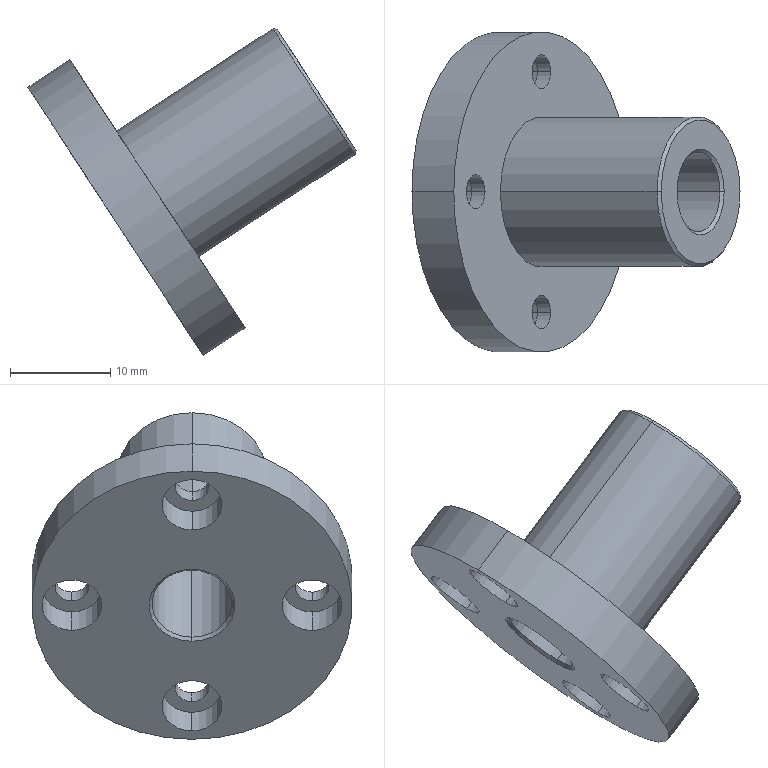Component | SolidWorks | LMF8UULinearBearing-1 | 1 solid | 35 faces | box 32.78 x 32 x 32.64 mm | volume 5725 mm3 | cylinder 22 | plane 7 | cone 6 | commonest cylinder face diameters 6 x8 3.4 x8 32 x2 8 x2 15 x2
STEP:
#1=COLOUR_RGB('',0.7922,0.8196,0.9333);
#2=FILL_AREA_STYLE_COLOUR('',#1);
#3=FILL_AREA_STYLE('',(#2));
#4=SURFACE_STYLE_FILL_AREA(#3);
#5=SURFACE_SIDE_STYLE('',(#4));
#6=SURFACE_STYLE_USAGE(.BOTH.,#5);
#7=PRESENTATION_STYLE_ASSIGNMENT((#6));
#8=CARTESIAN_POINT('',(-0.8628,2.344,0.7729));
#9=VERTEX_POINT('',#8);
#10=CARTESIAN_POINT('',(-0.6905,2.344,0.5092));
#11=VERTEX_POINT('',#10);
#12=CARTESIAN_POINT('',(-0.7767,2.344,0.6411));
#13=DIRECTION('',(0.8371,-0.,0.5471));
#14=DIRECTION('',(-0.5471,-0.0005991,0.8371));
#15=AXIS2_PLACEMENT_3D('',#12,#13,#14);
#16=CIRCLE('',#15,0.1575);
#17=EDGE_CURVE('',#9,#11,#16,.T.);
#18=ORIENTED_EDGE('',*,*,#17,.F.);
#19=CARTESIAN_POINT('',(-0.8594,2.344,0.7892));
#20=VERTEX_POINT('',#19);
#21=CARTESIAN_POINT('',(-0.8594,2.344,0.7892));
#22=DIRECTION('',(0.2051,-0.0004236,0.9787));
#23=VECTOR('',#22,39.37);
#24=LINE('',#21,#23);
#25=EDGE_CURVE('',#9,#20,#24,.T.);
#26=ORIENTED_EDGE('',*,*,#25,.T.);
#27=CARTESIAN_POINT('',(-0.6742,2.344,0.5058));
#28=VERTEX_POINT('',#27);
#29=CARTESIAN_POINT('',(-0.7668,2.344,0.6475));
#30=DIRECTION('',(-0.8371,0.,-0.5471));
#31=DIRECTION('',(-0.5471,-0.0005991,0.8371));
#32=AXIS2_PLACEMENT_3D('',#29,#30,#31);
#33=CIRCLE('',#32,0.1693);
#34=EDGE_CURVE('',#28,#20,#33,.T.);
#35=ORIENTED_EDGE('',*,*,#34,.F.);
#36=CARTESIAN_POINT('',(-0.6742,2.344,0.5058));
#37=DIRECTION('',(0.9787,0.0004236,-0.2051));
#38=VECTOR('',#37,39.37);
#39=LINE('',#36,#38);
#40=EDGE_CURVE('',#11,#28,#39,.T.);
#41=ORIENTED_EDGE('',*,*,#40,.F.);
#42=EDGE_LOOP('',(#18,#26,#35,#41));
#43=FACE_OUTER_BOUND('',#42,.T.);
#44=CARTESIAN_POINT('',(-0.7668,2.344,0.6475));
#45=DIRECTION('',(0.8371,-0.,0.5471));
#46=DIRECTION('',(0.5471,0.0005991,-0.8371));
#47=AXIS2_PLACEMENT_3D('',#44,#45,#46);
#48=CONICAL_SURFACE('',#47,0.1693,0.7854);
#49=ADVANCED_FACE('',(#43),#48,.F.);
#50=CARTESIAN_POINT('',(-0.6117,2.344,0.4102));
#51=VERTEX_POINT('',#50);
#52=CARTESIAN_POINT('',(-0.9219,2.344,0.8848));
#53=VERTEX_POINT('',#52);
#54=CARTESIAN_POINT('',(-0.7668,2.344,0.6475));
#55=DIRECTION('',(0.8371,-0.,0.5471));
#56=DIRECTION('',(-0.5471,-0.0005991,0.8371));
#57=AXIS2_PLACEMENT_3D('',#54,#55,#56);
#58=CIRCLE('',#57,0.2835);
#59=EDGE_CURVE('',#51,#53,#58,.T.);
#60=ORIENTED_EDGE('',*,*,#59,.F.);
#61=CARTESIAN_POINT('',(-0.6152,2.344,0.3939));
#62=VERTEX_POINT('',#61);
#63=CARTESIAN_POINT('',(-0.6152,2.344,0.3939));
#64=DIRECTION('',(-0.2051,0.0004236,-0.9787));
#65=VECTOR('',#64,39.37);
#66=LINE('',#63,#65);
#67=EDGE_CURVE('',#51,#62,#66,.T.);
#68=ORIENTED_EDGE('',*,*,#67,.T.);
#69=CARTESIAN_POINT('',(-0.9382,2.344,0.8882));
#70=VERTEX_POINT('',#69);
#71=CARTESIAN_POINT('',(-0.7767,2.344,0.6411));
#72=DIRECTION('',(-0.8371,0.,-0.5471));
#73=DIRECTION('',(-0.5471,-0.0005991,0.8371));
#74=AXIS2_PLACEMENT_3D('',#71,#72,#73);
#75=CIRCLE('',#74,0.2953);
#76=EDGE_CURVE('',#70,#62,#75,.T.);
#77=ORIENTED_EDGE('',*,*,#76,.F.);
#78=CARTESIAN_POINT('',(-0.9382,2.344,0.8882));
#79=DIRECTION('',(-0.9787,-0.0004236,0.2051));
#80=VECTOR('',#79,39.37);
#81=LINE('',#78,#80);
#82=EDGE_CURVE('',#53,#70,#81,.T.);
#83=ORIENTED_EDGE('',*,*,#82,.F.);
#84=EDGE_LOOP('',(#60,#68,#77,#83));
#85=FACE_OUTER_BOUND('',#84,.T.);
#86=CARTESIAN_POINT('',(-0.7767,2.344,0.6411));
#87=DIRECTION('',(-0.8371,0.,-0.5471));
#88=DIRECTION('',(-0.5471,-0.0005991,0.8371));
#89=AXIS2_PLACEMENT_3D('',#86,#87,#88);
#90=CONICAL_SURFACE('',#89,0.2953,0.7854);
#91=ADVANCED_FACE('',(#85),#90,.T.);
#92=CARTESIAN_POINT('',(-1.462,2.344,0.005266));
#93=VERTEX_POINT('',#92);
#94=CARTESIAN_POINT('',(-1.634,2.344,0.2689));
#95=VERTEX_POINT('',#94);
#96=CARTESIAN_POINT('',(-1.548,2.344,0.1371));
#97=DIRECTION('',(-0.8371,0.,-0.5471));
#98=DIRECTION('',(-0.5471,-0.0005991,0.8371));
#99=AXIS2_PLACEMENT_3D('',#96,#97,#98);
#100=CIRCLE('',#99,0.1575);
#101=EDGE_CURVE('',#93,#95,#100,.T.);
#102=ORIENTED_EDGE('',*,*,#101,.F.);
#103=CARTESIAN_POINT('',(-1.465,2.344,-0.01108));
#104=VERTEX_POINT('',#103);
#105=CARTESIAN_POINT('',(-1.462,2.344,0.005266));
#106=DIRECTION('',(-0.2051,0.0004236,-0.9787));
#107=VECTOR('',#106,39.37);
#108=LINE('',#105,#107);
#109=EDGE_CURVE('',#93,#104,#108,.T.);
#110=ORIENTED_EDGE('',*,*,#109,.T.);
#111=CARTESIAN_POINT('',(-1.65,2.344,0.2723));
#112=VERTEX_POINT('',#111);
#113=CARTESIAN_POINT('',(-1.558,2.344,0.1306));
#114=DIRECTION('',(0.8371,-0.,0.5471));
#115=DIRECTION('',(-0.5471,-0.0005991,0.8371));
#116=AXIS2_PLACEMENT_3D('',#113,#114,#115);
#117=CIRCLE('',#116,0.1693);
#118=EDGE_CURVE('',#112,#104,#117,.T.);
#119=ORIENTED_EDGE('',*,*,#118,.F.);
#120=CARTESIAN_POINT('',(-1.634,2.344,0.2689));
#121=DIRECTION('',(-0.9787,-0.0004236,0.2051));
#122=VECTOR('',#121,39.37);
#123=LINE('',#120,#122);
#124=EDGE_CURVE('',#95,#112,#123,.T.);
#125=ORIENTED_EDGE('',*,*,#124,.F.);
#126=EDGE_LOOP('',(#102,#110,#119,#125));
#127=FACE_OUTER_BOUND('',#126,.T.);
#128=CARTESIAN_POINT('',(-1.548,2.344,0.1371));
#129=DIRECTION('',(-0.8371,0.,-0.5471));
#130=DIRECTION('',(-0.5471,-0.0005991,0.8371));
#131=AXIS2_PLACEMENT_3D('',#128,#129,#130);
#132=CONICAL_SURFACE('',#131,0.1575,0.7854);
#133=ADVANCED_FACE('',(#127),#132,.F.);
#134=CARTESIAN_POINT('',(-1.381,2.817,0.1052));
#135=VERTEX_POINT('',#134);
#136=CARTESIAN_POINT('',(-1.51,2.817,0.303));
#137=VERTEX_POINT('',#136);
#138=CARTESIAN_POINT('',(-1.446,2.817,0.2041));
#139=DIRECTION('',(-0.8371,0.,-0.5471));
#140=DIRECTION('',(-0.5471,-0.0005991,0.8371));
#141=AXIS2_PLACEMENT_3D('',#138,#139,#140);
#142=CIRCLE('',#141,0.1181);
#143=EDGE_CURVE('',#135,#137,#142,.T.);
#144=ORIENTED_EDGE('',*,*,#143,.F.);
#145=CARTESIAN_POINT('',(-1.493,2.817,0.032));
#146=VERTEX_POINT('',#145);
#147=CARTESIAN_POINT('',(-1.493,2.817,0.032));
#148=DIRECTION('',(-0.8371,0.,-0.5471));
#149=VECTOR('',#148,39.37);
#150=LINE('',#147,#149);
#151=EDGE_CURVE('',#135,#146,#150,.T.);
#152=ORIENTED_EDGE('',*,*,#151,.T.);
#153=CARTESIAN_POINT('',(-1.623,2.817,0.2297));
#154=VERTEX_POINT('',#153);
#155=CARTESIAN_POINT('',(-1.558,2.817,0.1309));
#156=DIRECTION('',(-0.8371,0.,-0.5471));
#157=DIRECTION('',(-0.5471,-0.0005991,0.8371));
#158=AXIS2_PLACEMENT_3D('',#155,#156,#157);
#159=CIRCLE('',#158,0.1181);
#160=EDGE_CURVE('',#146,#154,#159,.T.);
#161=ORIENTED_EDGE('',*,*,#160,.T.);
#162=CARTESIAN_POINT('',(-1.623,2.817,0.2297));
#163=DIRECTION('',(-0.8371,0.,-0.5471));
#164=VECTOR('',#163,39.37);
#165=LINE('',#162,#164);
#166=EDGE_CURVE('',#137,#154,#165,.T.);
#167=ORIENTED_EDGE('',*,*,#166,.F.);
#168=EDGE_LOOP('',(#144,#152,#161,#167));
#169=FACE_OUTER_BOUND('',#168,.T.);
#170=CARTESIAN_POINT('',(-1.558,2.817,0.1309));
#171=DIRECTION('',(-0.8371,0.,-0.5471));
#172=DIRECTION('',(-0.5471,-0.0005991,0.8371));
#173=AXIS2_PLACEMENT_3D('',#170,#171,#172);
#174=CYLINDRICAL_SURFACE('',#173,0.1181);
#175=ADVANCED_FACE('',(#169),#174,.F.);
#176=CARTESIAN_POINT('',(-1.357,2.817,0.1825));
#177=VERTEX_POINT('',#176);
#178=CARTESIAN_POINT('',(-1.43,2.817,0.2946));
#179=VERTEX_POINT('',#178);
#180=CARTESIAN_POINT('',(-1.393,2.817,0.2386));
#181=DIRECTION('',(-0.8371,0.,-0.5471));
#182=DIRECTION('',(-0.5471,-0.0005991,0.8371));
#183=AXIS2_PLACEMENT_3D('',#180,#181,#182);
#184=CIRCLE('',#183,0.06693);
#185=EDGE_CURVE('',#177,#179,#184,.T.);
#186=ORIENTED_EDGE('',*,*,#185,.F.);
#187=CARTESIAN_POINT('',(-1.409,2.817,0.1481));
#188=VERTEX_POINT('',#187);
#189=CARTESIAN_POINT('',(-1.521,2.817,0.07484));
#190=DIRECTION('',(-0.8371,0.,-0.5471));
#191=VECTOR('',#190,39.37);
#192=LINE('',#189,#191);
#193=EDGE_CURVE('',#177,#188,#192,.T.);
#194=ORIENTED_EDGE('',*,*,#193,.T.);
#195=CARTESIAN_POINT('',(-1.482,2.817,0.2601));
#196=VERTEX_POINT('',#195);
#197=CARTESIAN_POINT('',(-1.446,2.817,0.2041));
#198=DIRECTION('',(-0.8371,0.,-0.5471));
#199=DIRECTION('',(-0.5471,-0.0005991,0.8371));
#200=AXIS2_PLACEMENT_3D('',#197,#198,#199);
#201=CIRCLE('',#200,0.06693);
#202=EDGE_CURVE('',#188,#196,#201,.T.);
#203=ORIENTED_EDGE('',*,*,#202,.T.);
#204=CARTESIAN_POINT('',(-1.595,2.817,0.1869));
#205=DIRECTION('',(-0.8371,0.,-0.5471));
#206=VECTOR('',#205,39.37);
#207=LINE('',#204,#206);
#208=EDGE_CURVE('',#179,#196,#207,.T.);
#209=ORIENTED_EDGE('',*,*,#208,.F.);
#210=EDGE_LOOP('',(#186,#194,#203,#209));
#211=FACE_OUTER_BOUND('',#210,.T.);
#212=CARTESIAN_POINT('',(-1.558,2.817,0.1309));
#213=DIRECTION('',(-0.8371,0.,-0.5471));
#214=DIRECTION('',(-0.5471,-0.0005991,0.8371));
#215=AXIS2_PLACEMENT_3D('',#212,#213,#214);
#216=CYLINDRICAL_SURFACE('',#215,0.06693);
#217=ADVANCED_FACE('',(#211),#216,.F.);
#218=CARTESIAN_POINT('',(-1.123,2.345,-0.2905));
#219=VERTEX_POINT('',#218);
#220=CARTESIAN_POINT('',(-1.252,2.345,-0.09275));
#221=VERTEX_POINT('',#220);
#222=CARTESIAN_POINT('',(-1.187,2.345,-0.1916));
#223=DIRECTION('',(-0.8371,0.,-0.5471));
#224=DIRECTION('',(-0.5471,-0.0005991,0.8371));
#225=AXIS2_PLACEMENT_3D('',#222,#223,#224);
#226=CIRCLE('',#225,0.1181);
#227=EDGE_CURVE('',#219,#221,#226,.T.);
#228=ORIENTED_EDGE('',*,*,#227,.F.);
#229=CARTESIAN_POINT('',(-1.235,2.345,-0.3637));
#230=VERTEX_POINT('',#229);
#231=CARTESIAN_POINT('',(-1.235,2.345,-0.3637));
#232=DIRECTION('',(-0.8371,0.,-0.5471));
#233=VECTOR('',#232,39.37);
#234=LINE('',#231,#233);
#235=EDGE_CURVE('',#219,#230,#234,.T.);
#236=ORIENTED_EDGE('',*,*,#235,.T.);
#237=CARTESIAN_POINT('',(-1.364,2.345,-0.166));
#238=VERTEX_POINT('',#237);
#239=CARTESIAN_POINT('',(-1.299,2.345,-0.2648));
#240=DIRECTION('',(-0.8371,0.,-0.5471));
#241=DIRECTION('',(-0.5471,-0.0005991,0.8371));
#242=AXIS2_PLACEMENT_3D('',#239,#240,#241);
#243=CIRCLE('',#242,0.1181);
#244=EDGE_CURVE('',#230,#238,#243,.T.);
#245=ORIENTED_EDGE('',*,*,#244,.T.);
#246=CARTESIAN_POINT('',(-1.364,2.345,-0.166));
#247=DIRECTION('',(-0.8371,0.,-0.5471));
#248=VECTOR('',#247,39.37);
#249=LINE('',#246,#248);
#250=EDGE_CURVE('',#221,#238,#249,.T.);
#251=ORIENTED_EDGE('',*,*,#250,.F.);
#252=EDGE_LOOP('',(#228,#236,#245,#251));
#253=FACE_OUTER_BOUND('',#252,.T.);
#254=CARTESIAN_POINT('',(-1.299,2.345,-0.2648));
#255=DIRECTION('',(-0.8371,0.,-0.5471));
#256=DIRECTION('',(-0.5471,-0.0005991,0.8371));
#257=AXIS2_PLACEMENT_3D('',#254,#255,#256);
#258=CYLINDRICAL_SURFACE('',#257,0.1181);
#259=ADVANCED_FACE('',(#253),#258,.F.);
#260=CARTESIAN_POINT('',(-1.098,2.345,-0.2132));
#261=VERTEX_POINT('',#260);
#262=CARTESIAN_POINT('',(-1.171,2.345,-0.1011));
#263=VERTEX_POINT('',#262);
#264=CARTESIAN_POINT('',(-1.135,2.345,-0.1572));
#265=DIRECTION('',(-0.8371,0.,-0.5471));
#266=DIRECTION('',(-0.5471,-0.0005991,0.8371));
#267=AXIS2_PLACEMENT_3D('',#264,#265,#266);
#268=CIRCLE('',#267,0.06693);
#269=EDGE_CURVE('',#261,#263,#268,.T.);
#270=ORIENTED_EDGE('',*,*,#269,.F.);
#271=CARTESIAN_POINT('',(-1.151,2.345,-0.2476));
#272=VERTEX_POINT('',#271);
#273=CARTESIAN_POINT('',(-1.263,2.345,-0.3209));
#274=DIRECTION('',(-0.8371,0.,-0.5471));
#275=VECTOR('',#274,39.37);
#276=LINE('',#273,#275);
#277=EDGE_CURVE('',#261,#272,#276,.T.);
#278=ORIENTED_EDGE('',*,*,#277,.T.);
#279=CARTESIAN_POINT('',(-1.224,2.345,-0.1356));
#280=VERTEX_POINT('',#279);
#281=CARTESIAN_POINT('',(-1.187,2.345,-0.1916));
#282=DIRECTION('',(-0.8371,0.,-0.5471));
#283=DIRECTION('',(-0.5471,-0.0005991,0.8371));
#284=AXIS2_PLACEMENT_3D('',#281,#282,#283);
#285=CIRCLE('',#284,0.06693);
#286=EDGE_CURVE('',#272,#280,#285,.T.);
#287=ORIENTED_EDGE('',*,*,#286,.T.);
#288=CARTESIAN_POINT('',(-1.336,2.345,-0.2088));
#289=DIRECTION('',(-0.8371,0.,-0.5471));
#290=VECTOR('',#289,39.37);
#291=LINE('',#288,#290);
#292=EDGE_CURVE('',#263,#280,#291,.T.);
#293=ORIENTED_EDGE('',*,*,#292,.F.);
#294=EDGE_LOOP('',(#270,#278,#287,#293));
#295=FACE_OUTER_BOUND('',#294,.T.);
#296=CARTESIAN_POINT('',(-1.299,2.345,-0.2648));
#297=DIRECTION('',(-0.8371,0.,-0.5471));
#298=DIRECTION('',(-0.5471,-0.0005991,0.8371));
#299=AXIS2_PLACEMENT_3D('',#296,#297,#298);
#300=CYLINDRICAL_SURFACE('',#299,0.06693);
#301=ADVANCED_FACE('',(#295),#300,.F.);
#302=CARTESIAN_POINT('',(-1.381,1.872,0.1048));
#303=VERTEX_POINT('',#302);
#304=CARTESIAN_POINT('',(-1.51,1.872,0.3025));
#305=VERTEX_POINT('',#304);
#306=CARTESIAN_POINT('',(-1.446,1.872,0.2036));
#307=DIRECTION('',(-0.8371,0.,-0.5471));
#308=DIRECTION('',(-0.5471,-0.0005991,0.8371));
#309=AXIS2_PLACEMENT_3D('',#306,#307,#308);
#310=CIRCLE('',#309,0.1181);
#311=EDGE_CURVE('',#303,#305,#310,.T.);
#312=ORIENTED_EDGE('',*,*,#311,.F.);
#313=CARTESIAN_POINT('',(-1.493,1.872,0.03152));
#314=VERTEX_POINT('',#313);
#315=CARTESIAN_POINT('',(-1.493,1.872,0.03152));
#316=DIRECTION('',(-0.8371,0.,-0.5471));
#317=VECTOR('',#316,39.37);
#318=LINE('',#315,#317);
#319=EDGE_CURVE('',#303,#314,#318,.T.);
#320=ORIENTED_EDGE('',*,*,#319,.T.);
#321=CARTESIAN_POINT('',(-1.622,1.872,0.2293));
#322=VERTEX_POINT('',#321);
#323=CARTESIAN_POINT('',(-1.558,1.872,0.1304));
#324=DIRECTION('',(-0.8371,0.,-0.5471));
#325=DIRECTION('',(-0.5471,-0.0005991,0.8371));
#326=AXIS2_PLACEMENT_3D('',#323,#324,#325);
#327=CIRCLE('',#326,0.1181);
#328=EDGE_CURVE('',#314,#322,#327,.T.);
#329=ORIENTED_EDGE('',*,*,#328,.T.);
#330=CARTESIAN_POINT('',(-1.622,1.872,0.2293));
#331=DIRECTION('',(-0.8371,0.,-0.5471));
#332=VECTOR('',#331,39.37);
#333=LINE('',#330,#332);
#334=EDGE_CURVE('',#305,#322,#333,.T.);
#335=ORIENTED_EDGE('',*,*,#334,.F.);
#336=EDGE_LOOP('',(#312,#320,#329,#335));
#337=FACE_OUTER_BOUND('',#336,.T.);
#338=CARTESIAN_POINT('',(-1.558,1.872,0.1304));
#339=DIRECTION('',(-0.8371,0.,-0.5471));
#340=DIRECTION('',(-0.5471,-0.0005991,0.8371));
#341=AXIS2_PLACEMENT_3D('',#338,#339,#340);
#342=CYLINDRICAL_SURFACE('',#341,0.1181);
#343=ADVANCED_FACE('',(#337),#342,.F.);
#344=CARTESIAN_POINT('',(-1.356,1.872,0.1821));
#345=VERTEX_POINT('',#344);
#346=CARTESIAN_POINT('',(-1.429,1.872,0.2941));
#347=VERTEX_POINT('',#346);
#348=CARTESIAN_POINT('',(-1.393,1.872,0.2381));
#349=DIRECTION('',(-0.8371,0.,-0.5471));
#350=DIRECTION('',(-0.5471,-0.0005991,0.8371));
#351=AXIS2_PLACEMENT_3D('',#348,#349,#350);
#352=CIRCLE('',#351,0.06693);
#353=EDGE_CURVE('',#345,#347,#352,.T.);
#354=ORIENTED_EDGE('',*,*,#353,.F.);
#355=CARTESIAN_POINT('',(-1.409,1.872,0.1476));
#356=VERTEX_POINT('',#355);
#357=CARTESIAN_POINT('',(-1.521,1.872,0.07437));
#358=DIRECTION('',(-0.8371,0.,-0.5471));
#359=VECTOR('',#358,39.37);
#360=LINE('',#357,#359);
#361=EDGE_CURVE('',#345,#356,#360,.T.);
#362=ORIENTED_EDGE('',*,*,#361,.T.);
#363=CARTESIAN_POINT('',(-1.482,1.872,0.2596));
#364=VERTEX_POINT('',#363);
#365=CARTESIAN_POINT('',(-1.446,1.872,0.2036));
#366=DIRECTION('',(-0.8371,0.,-0.5471));
#367=DIRECTION('',(-0.5471,-0.0005991,0.8371));
#368=AXIS2_PLACEMENT_3D('',#365,#366,#367);
#369=CIRCLE('',#368,0.06693);
#370=EDGE_CURVE('',#356,#364,#369,.T.);
#371=ORIENTED_EDGE('',*,*,#370,.T.);
#372=CARTESIAN_POINT('',(-1.594,1.872,0.1864));
#373=DIRECTION('',(-0.8371,0.,-0.5471));
#374=VECTOR('',#373,39.37);
#375=LINE('',#372,#374);
#376=EDGE_CURVE('',#347,#364,#375,.T.);
#377=ORIENTED_EDGE('',*,*,#376,.F.);
#378=EDGE_LOOP('',(#354,#362,#371,#377));
#379=FACE_OUTER_BOUND('',#378,.T.);
#380=CARTESIAN_POINT('',(-1.558,1.872,0.1304));
#381=DIRECTION('',(-0.8371,0.,-0.5471));
#382=DIRECTION('',(-0.5471,-0.0005991,0.8371));
#383=AXIS2_PLACEMENT_3D('',#380,#381,#382);
#384=CYLINDRICAL_SURFACE('',#383,0.06693);
#385=ADVANCED_FACE('',(#379),#384,.F.);
#386=CARTESIAN_POINT('',(-1.64,2.344,0.5005));
#387=VERTEX_POINT('',#386);
#388=CARTESIAN_POINT('',(-1.769,2.344,0.6982));
#389=VERTEX_POINT('',#388);
#390=CARTESIAN_POINT('',(-1.704,2.344,0.5993));
#391=DIRECTION('',(-0.8371,0.,-0.5471));
#392=DIRECTION('',(-0.5471,-0.0005991,0.8371));
#393=AXIS2_PLACEMENT_3D('',#390,#391,#392);
#394=CIRCLE('',#393,0.1181);
#395=EDGE_CURVE('',#387,#389,#394,.T.);
#396=ORIENTED_EDGE('',*,*,#395,.F.);
#397=CARTESIAN_POINT('',(-1.752,2.344,0.4272));
#398=VERTEX_POINT('',#397);
#399=CARTESIAN_POINT('',(-1.752,2.344,0.4272));
#400=DIRECTION('',(-0.8371,0.,-0.5471));
#401=VECTOR('',#400,39.37);
#402=LINE('',#399,#401);
#403=EDGE_CURVE('',#387,#398,#402,.T.);
#404=ORIENTED_EDGE('',*,*,#403,.T.);
#405=CARTESIAN_POINT('',(-1.881,2.344,0.625));
#406=VERTEX_POINT('',#405);
#407=CARTESIAN_POINT('',(-1.816,2.344,0.5261));
#408=DIRECTION('',(-0.8371,0.,-0.5471));
#409=DIRECTION('',(-0.5471,-0.0005991,0.8371));
#410=AXIS2_PLACEMENT_3D('',#407,#408,#409);
#411=CIRCLE('',#410,0.1181);
#412=EDGE_CURVE('',#398,#406,#411,.T.);
#413=ORIENTED_EDGE('',*,*,#412,.T.);
#414=CARTESIAN_POINT('',(-1.881,2.344,0.625));
#415=DIRECTION('',(-0.8371,0.,-0.5471));
#416=VECTOR('',#415,39.37);
#417=LINE('',#414,#416);
#418=EDGE_CURVE('',#389,#406,#417,.T.);
#419=ORIENTED_EDGE('',*,*,#418,.F.);
#420=EDGE_LOOP('',(#396,#404,#413,#419));
#421=FACE_OUTER_BOUND('',#420,.T.);
#422=CARTESIAN_POINT('',(-1.816,2.344,0.5261));
#423=DIRECTION('',(-0.8371,0.,-0.5471));
#424=DIRECTION('',(-0.5471,-0.0005991,0.8371));
#425=AXIS2_PLACEMENT_3D('',#422,#423,#424);
#426=CYLINDRICAL_SURFACE('',#425,0.1181);
#427=ADVANCED_FACE('',(#421),#426,.F.);
#428=CARTESIAN_POINT('',(-1.615,2.344,0.5778));
#429=VERTEX_POINT('',#428);
#430=CARTESIAN_POINT('',(-1.688,2.344,0.6898));
#431=VERTEX_POINT('',#430);
#432=CARTESIAN_POINT('',(-1.651,2.344,0.6338));
#433=DIRECTION('',(-0.8371,0.,-0.5471));
#434=DIRECTION('',(-0.5471,-0.0005991,0.8371));
#435=AXIS2_PLACEMENT_3D('',#432,#433,#434);
#436=CIRCLE('',#435,0.06693);
#437=EDGE_CURVE('',#429,#431,#436,.T.);
#438=ORIENTED_EDGE('',*,*,#437,.F.);
#439=CARTESIAN_POINT('',(-1.668,2.344,0.5433));
#440=VERTEX_POINT('',#439);
#441=CARTESIAN_POINT('',(-1.78,2.344,0.4701));
#442=DIRECTION('',(-0.8371,0.,-0.5471));
#443=VECTOR('',#442,39.37);
#444=LINE('',#441,#443);
#445=EDGE_CURVE('',#429,#440,#444,.T.);
#446=ORIENTED_EDGE('',*,*,#445,.T.);
#447=CARTESIAN_POINT('',(-1.741,2.344,0.6554));
#448=VERTEX_POINT('',#447);
#449=CARTESIAN_POINT('',(-1.704,2.344,0.5993));
#450=DIRECTION('',(-0.8371,0.,-0.5471));
#451=DIRECTION('',(-0.5471,-0.0005991,0.8371));
#452=AXIS2_PLACEMENT_3D('',#449,#450,#451);
#453=CIRCLE('',#452,0.06693);
#454=EDGE_CURVE('',#440,#448,#453,.T.);
#455=ORIENTED_EDGE('',*,*,#454,.T.);
#456=CARTESIAN_POINT('',(-1.853,2.344,0.5821));
#457=DIRECTION('',(-0.8371,0.,-0.5471));
#458=VECTOR('',#457,39.37);
#459=LINE('',#456,#458);
#460=EDGE_CURVE('',#431,#448,#459,.T.);
#461=ORIENTED_EDGE('',*,*,#460,.F.);
#462=EDGE_LOOP('',(#438,#446,#455,#461));
#463=FACE_OUTER_BOUND('',#462,.T.);
#464=CARTESIAN_POINT('',(-1.816,2.344,0.5261));
#465=DIRECTION('',(-0.8371,0.,-0.5471));
#466=DIRECTION('',(-0.5471,-0.0005991,0.8371));
#467=AXIS2_PLACEMENT_3D('',#464,#465,#466);
#468=CYLINDRICAL_SURFACE('',#467,0.06693);
#469=ADVANCED_FACE('',(#463),#468,.F.);
#470=CARTESIAN_POINT('',(-1.902,2.344,0.6579));
#471=VERTEX_POINT('',#470);
#472=CARTESIAN_POINT('',(-1.213,2.345,-0.3967));
#473=VERTEX_POINT('',#472);
#474=CARTESIAN_POINT('',(-1.558,2.344,0.1306));
#475=DIRECTION('',(-0.8371,0.,-0.5471));
#476=DIRECTION('',(-0.5471,-0.0005991,0.8371));
#477=AXIS2_PLACEMENT_3D('',#474,#475,#476);
#478=CIRCLE('',#477,0.6299);
#479=EDGE_CURVE('',#471,#473,#478,.T.);
#480=ORIENTED_EDGE('',*,*,#479,.F.);
#481=CARTESIAN_POINT('',(-1.738,2.344,0.7656));
#482=VERTEX_POINT('',#481);
#483=CARTESIAN_POINT('',(-1.902,2.344,0.6579));
#484=DIRECTION('',(0.8371,-0.,0.5471));
#485=VECTOR('',#484,39.37);
#486=LINE('',#483,#485);
#487=EDGE_CURVE('',#471,#482,#486,.T.);
#488=ORIENTED_EDGE('',*,*,#487,.T.);
#489=CARTESIAN_POINT('',(-1.048,2.345,-0.289));
#490=VERTEX_POINT('',#489);
#491=CARTESIAN_POINT('',(-1.393,2.344,0.2383));
#492=DIRECTION('',(-0.8371,0.,-0.5471));
#493=DIRECTION('',(-0.5471,-0.0005991,0.8371));
#494=AXIS2_PLACEMENT_3D('',#491,#492,#493);
#495=CIRCLE('',#494,0.6299);
#496=EDGE_CURVE('',#482,#490,#495,.T.);
#497=ORIENTED_EDGE('',*,*,#496,.T.);
#498=CARTESIAN_POINT('',(-1.213,2.345,-0.3967));
#499=DIRECTION('',(0.8371,-0.,0.5471));
#500=VECTOR('',#499,39.37);
#501=LINE('',#498,#500);
#502=EDGE_CURVE('',#473,#490,#501,.T.);
#503=ORIENTED_EDGE('',*,*,#502,.F.);
#504=EDGE_LOOP('',(#480,#488,#497,#503));
#505=FACE_OUTER_BOUND('',#504,.T.);
#506=CARTESIAN_POINT('',(-1.558,2.344,0.1306));
#507=DIRECTION('',(0.8371,-0.,0.5471));
#508=DIRECTION('',(0.5471,0.0005991,-0.8371));
#509=AXIS2_PLACEMENT_3D('',#506,#507,#508);
#510=CYLINDRICAL_SURFACE('',#509,0.6299);
#511=ADVANCED_FACE('',(#505),#510,.T.);
#512=ORIENTED_EDGE('',*,*,#101,.T.);
#513=CARTESIAN_POINT('',(-1.479,2.344,0.3701));
#514=DIRECTION('',(0.8371,-0.,0.5471));
#515=VECTOR('',#514,39.37);
#516=LINE('',#513,#515);
#517=EDGE_CURVE('',#95,#9,#516,.T.);
#518=ORIENTED_EDGE('',*,*,#517,.T.);
#519=ORIENTED_EDGE('',*,*,#17,.T.);
#520=CARTESIAN_POINT('',(-1.307,2.344,0.1065));
#521=DIRECTION('',(0.8371,-0.,0.5471));
#522=VECTOR('',#521,39.37);
#523=LINE('',#520,#522);
#524=EDGE_CURVE('',#93,#11,#523,.T.);
#525=ORIENTED_EDGE('',*,*,#524,.F.);
#526=EDGE_LOOP('',(#512,#518,#519,#525));
#527=FACE_OUTER_BOUND('',#526,.T.);
#528=CARTESIAN_POINT('',(-1.393,2.344,0.2383));
#529=DIRECTION('',(0.8371,-0.,0.5471));
#530=DIRECTION('',(0.5471,0.0005991,-0.8371));
#531=AXIS2_PLACEMENT_3D('',#528,#529,#530);
#532=CYLINDRICAL_SURFACE('',#531,0.1575);
#533=ADVANCED_FACE('',(#527),#532,.F.);
#534=CARTESIAN_POINT('',(-1.555,2.344,0.4855));
#535=VERTEX_POINT('',#534);
#536=CARTESIAN_POINT('',(-1.231,2.344,-0.008856));
#537=VERTEX_POINT('',#536);
#538=CARTESIAN_POINT('',(-1.393,2.344,0.2383));
#539=DIRECTION('',(-0.8371,0.,-0.5471));
#540=DIRECTION('',(-0.5471,-0.0005991,0.8371));
#541=AXIS2_PLACEMENT_3D('',#538,#539,#540);
#542=CIRCLE('',#541,0.2953);
#543=EDGE_CURVE('',#535,#537,#542,.T.);
#544=ORIENTED_EDGE('',*,*,#543,.F.);
#545=CARTESIAN_POINT('',(-1.555,2.344,0.4855));
#546=DIRECTION('',(0.8371,-0.,0.5471));
#547=VECTOR('',#546,39.37);
#548=LINE('',#545,#547);
#549=EDGE_CURVE('',#535,#70,#548,.T.);
#550=ORIENTED_EDGE('',*,*,#549,.T.);
#551=ORIENTED_EDGE('',*,*,#76,.T.);
#552=CARTESIAN_POINT('',(-1.231,2.344,-0.008856));
#553=DIRECTION('',(0.8371,-0.,0.5471));
#554=VECTOR('',#553,39.37);
#555=LINE('',#552,#554);
#556=EDGE_CURVE('',#537,#62,#555,.T.);
#557=ORIENTED_EDGE('',*,*,#556,.F.);
#558=EDGE_LOOP('',(#544,#550,#551,#557));
#559=FACE_OUTER_BOUND('',#558,.T.);
#560=CARTESIAN_POINT('',(-1.393,2.344,0.2383));
#561=DIRECTION('',(0.8371,-0.,0.5471));
#562=DIRECTION('',(0.5471,0.0005991,-0.8371));
#563=AXIS2_PLACEMENT_3D('',#560,#561,#562);
#564=CYLINDRICAL_SURFACE('',#563,0.2953);
#565=ADVANCED_FACE('',(#559),#564,.T.);
#566=CARTESIAN_POINT('',(-0.7668,2.344,0.6475));
#567=DIRECTION('',(0.8371,-0.,0.5471));
#568=DIRECTION('',(-0.5471,-0.0005991,0.8371));
#569=AXIS2_PLACEMENT_3D('',#566,#567,#568);
#570=CIRCLE('',#569,0.2835);
#571=EDGE_CURVE('',#53,#51,#570,.T.);
#572=ORIENTED_EDGE('',*,*,#571,.T.);
#573=ORIENTED_EDGE('',*,*,#59,.T.);
#574=EDGE_LOOP('',(#572,#573));
#575=FACE_OUTER_BOUND('',#574,.T.);
#576=ORIENTED_EDGE('',*,*,#34,.T.);
#577=CARTESIAN_POINT('',(-0.7668,2.344,0.6475));
#578=DIRECTION('',(-0.8371,0.,-0.5471));
#579=DIRECTION('',(-0.5471,-0.0005991,0.8371));
#580=AXIS2_PLACEMENT_3D('',#577,#578,#579);
#581=CIRCLE('',#580,0.1693);
#582=EDGE_CURVE('',#20,#28,#581,.T.);
#583=ORIENTED_EDGE('',*,*,#582,.T.);
#584=EDGE_LOOP('',(#576,#583));
#585=FACE_BOUND('',#584,.T.);
#586=CARTESIAN_POINT('',(-0.7668,2.344,0.6475));
#587=DIRECTION('',(-0.8371,0.,-0.5471));
#588=DIRECTION('',(-0.5471,-0.0005991,0.8371));
#589=AXIS2_PLACEMENT_3D('',#586,#587,#588);
#590=PLANE('',#589);
#591=ADVANCED_FACE('',(#575,#585),#590,.F.);
#592=ORIENTED_EDGE('',*,*,#549,.F.);
#593=CARTESIAN_POINT('',(-1.393,2.344,0.2383));
#594=DIRECTION('',(-0.8371,0.,-0.5471));
#595=DIRECTION('',(-0.5471,-0.0005991,0.8371));
#596=AXIS2_PLACEMENT_3D('',#593,#594,#595);
#597=CIRCLE('',#596,0.2953);
#598=EDGE_CURVE('',#537,#535,#597,.T.);
#599=ORIENTED_EDGE('',*,*,#598,.F.);
#600=ORIENTED_EDGE('',*,*,#556,.T.);
#601=CARTESIAN_POINT('',(-0.7767,2.344,0.6411));
#602=DIRECTION('',(-0.8371,0.,-0.5471));
#603=DIRECTION('',(-0.5471,-0.0005991,0.8371));
#604=AXIS2_PLACEMENT_3D('',#601,#602,#603);
#605=CIRCLE('',#604,0.2953);
#606=EDGE_CURVE('',#62,#70,#605,.T.);
#607=ORIENTED_EDGE('',*,*,#606,.T.);
#608=EDGE_LOOP('',(#592,#599,#600,#607));
#609=FACE_OUTER_BOUND('',#608,.T.);
#610=CARTESIAN_POINT('',(-1.393,2.344,0.2383));
#611=DIRECTION('',(0.8371,-0.,0.5471));
#612=DIRECTION('',(0.5471,0.0005991,-0.8371));
#613=AXIS2_PLACEMENT_3D('',#610,#611,#612);
#614=CYLINDRICAL_SURFACE('',#613,0.2953);
#615=ADVANCED_FACE('',(#609),#614,.T.);
#616=ORIENTED_EDGE('',*,*,#517,.F.);
#617=CARTESIAN_POINT('',(-1.548,2.344,0.1371));
#618=DIRECTION('',(-0.8371,0.,-0.5471));
#619=DIRECTION('',(-0.5471,-0.0005991,0.8371));
#620=AXIS2_PLACEMENT_3D('',#617,#618,#619);
#621=CIRCLE('',#620,0.1575);
#622=EDGE_CURVE('',#95,#93,#621,.T.);
#623=ORIENTED_EDGE('',*,*,#622,.T.);
#624=ORIENTED_EDGE('',*,*,#524,.T.);
#625=CARTESIAN_POINT('',(-0.7767,2.344,0.6411));
#626=DIRECTION('',(0.8371,-0.,0.5471));
#627=DIRECTION('',(-0.5471,-0.0005991,0.8371));
#628=AXIS2_PLACEMENT_3D('',#625,#626,#627);
#629=CIRCLE('',#628,0.1575);
#630=EDGE_CURVE('',#11,#9,#629,.T.);
#631=ORIENTED_EDGE('',*,*,#630,.T.);
#632=EDGE_LOOP('',(#616,#623,#624,#631));
#633=FACE_OUTER_BOUND('',#632,.T.);
#634=CARTESIAN_POINT('',(-1.393,2.344,0.2383));
#635=DIRECTION('',(0.8371,-0.,0.5471));
#636=DIRECTION('',(0.5471,0.0005991,-0.8371));
#637=AXIS2_PLACEMENT_3D('',#634,#635,#636);
#638=CYLINDRICAL_SURFACE('',#637,0.1575);
#639=ADVANCED_FACE('',(#633),#638,.F.);
#640=CARTESIAN_POINT('',(-1.393,2.817,0.2386));
#641=DIRECTION('',(-0.8371,0.,-0.5471));
#642=DIRECTION('',(-0.5471,-0.0005991,0.8371));
#643=AXIS2_PLACEMENT_3D('',#640,#641,#642);
#644=CIRCLE('',#643,0.06693);
#645=EDGE_CURVE('',#179,#177,#644,.T.);
#646=ORIENTED_EDGE('',*,*,#645,.T.);
#647=ORIENTED_EDGE('',*,*,#185,.T.);
#648=EDGE_LOOP('',(#646,#647));
#649=FACE_BOUND('',#648,.T.);
#650=CARTESIAN_POINT('',(-1.135,2.345,-0.1572));
#651=DIRECTION('',(-0.8371,0.,-0.5471));
#652=DIRECTION('',(-0.5471,-0.0005991,0.8371));
#653=AXIS2_PLACEMENT_3D('',#650,#651,#652);
#654=CIRCLE('',#653,0.06693);
#655=EDGE_CURVE('',#263,#261,#654,.T.);
#656=ORIENTED_EDGE('',*,*,#655,.T.);
#657=ORIENTED_EDGE('',*,*,#269,.T.);
#658=EDGE_LOOP('',(#656,#657));
#659=FACE_BOUND('',#658,.T.);
#660=CARTESIAN_POINT('',(-1.393,1.872,0.2381));
#661=DIRECTION('',(-0.8371,0.,-0.5471));
#662=DIRECTION('',(-0.5471,-0.0005991,0.8371));
#663=AXIS2_PLACEMENT_3D('',#660,#661,#662);
#664=CIRCLE('',#663,0.06693);
#665=EDGE_CURVE('',#347,#345,#664,.T.);
#666=ORIENTED_EDGE('',*,*,#665,.T.);
#667=ORIENTED_EDGE('',*,*,#353,.T.);
#668=EDGE_LOOP('',(#666,#667));
#669=FACE_BOUND('',#668,.T.);
#670=CARTESIAN_POINT('',(-1.651,2.344,0.6338));
#671=DIRECTION('',(-0.8371,0.,-0.5471));
#672=DIRECTION('',(-0.5471,-0.0005991,0.8371));
#673=AXIS2_PLACEMENT_3D('',#670,#671,#672);
#674=CIRCLE('',#673,0.06693);
#675=EDGE_CURVE('',#431,#429,#674,.T.);
#676=ORIENTED_EDGE('',*,*,#675,.T.);
#677=ORIENTED_EDGE('',*,*,#437,.T.);
#678=EDGE_LOOP('',(#676,#677));
#679=FACE_BOUND('',#678,.T.);
#680=CARTESIAN_POINT('',(-1.393,2.344,0.2383));
#681=DIRECTION('',(-0.8371,0.,-0.5471));
#682=DIRECTION('',(-0.5471,-0.0005991,0.8371));
#683=AXIS2_PLACEMENT_3D('',#680,#681,#682);
#684=CIRCLE('',#683,0.6299);
#685=EDGE_CURVE('',#490,#482,#684,.T.);
#686=ORIENTED_EDGE('',*,*,#685,.F.);
#687=ORIENTED_EDGE('',*,*,#496,.F.);
#688=EDGE_LOOP('',(#686,#687));
#689=FACE_OUTER_BOUND('',#688,.T.);
#690=ORIENTED_EDGE('',*,*,#598,.T.);
#691=ORIENTED_EDGE('',*,*,#543,.T.);
#692=EDGE_LOOP('',(#690,#691));
#693=FACE_BOUND('',#692,.T.);
#694=CARTESIAN_POINT('',(-1.393,2.344,0.2383));
#695=DIRECTION('',(-0.8371,0.,-0.5471));
#696=DIRECTION('',(-0.5471,-0.0005991,0.8371));
#697=AXIS2_PLACEMENT_3D('',#694,#695,#696);
#698=PLANE('',#697);
#699=ADVANCED_FACE('',(#649,#659,#669,#679,#689,#693),#698,.F.);
#700=ORIENTED_EDGE('',*,*,#118,.T.);
#701=CARTESIAN_POINT('',(-1.558,2.344,0.1306));
#702=DIRECTION('',(0.8371,-0.,0.5471));
#703=DIRECTION('',(-0.5471,-0.0005991,0.8371));
#704=AXIS2_PLACEMENT_3D('',#701,#702,#703);
#705=CIRCLE('',#704,0.1693);
#706=EDGE_CURVE('',#104,#112,#705,.T.);
#707=ORIENTED_EDGE('',*,*,#706,.T.);
#708=EDGE_LOOP('',(#700,#707));
#709=FACE_BOUND('',#708,.T.);
#710=CARTESIAN_POINT('',(-1.558,2.817,0.1309));
#711=DIRECTION('',(-0.8371,0.,-0.5471));
#712=DIRECTION('',(-0.5471,-0.0005991,0.8371));
#713=AXIS2_PLACEMENT_3D('',#710,#711,#712);
#714=CIRCLE('',#713,0.1181);
#715=EDGE_CURVE('',#154,#146,#714,.T.);
#716=ORIENTED_EDGE('',*,*,#715,.F.);
#717=ORIENTED_EDGE('',*,*,#160,.F.);
#718=EDGE_LOOP('',(#716,#717));
#719=FACE_BOUND('',#718,.T.);
#720=CARTESIAN_POINT('',(-1.299,2.345,-0.2648));
#721=DIRECTION('',(-0.8371,0.,-0.5471));
#722=DIRECTION('',(-0.5471,-0.0005991,0.8371));
#723=AXIS2_PLACEMENT_3D('',#720,#721,#722);
#724=CIRCLE('',#723,0.1181);
#725=EDGE_CURVE('',#238,#230,#724,.T.);
#726=ORIENTED_EDGE('',*,*,#725,.F.);
#727=ORIENTED_EDGE('',*,*,#244,.F.);
#728=EDGE_LOOP('',(#726,#727));
#729=FACE_BOUND('',#728,.T.);
#730=CARTESIAN_POINT('',(-1.558,1.872,0.1304));
#731=DIRECTION('',(-0.8371,0.,-0.5471));
#732=DIRECTION('',(-0.5471,-0.0005991,0.8371));
#733=AXIS2_PLACEMENT_3D('',#730,#731,#732);
#734=CIRCLE('',#733,0.1181);
#735=EDGE_CURVE('',#322,#314,#734,.T.);
#736=ORIENTED_EDGE('',*,*,#735,.F.);
#737=ORIENTED_EDGE('',*,*,#328,.F.);
#738=EDGE_LOOP('',(#736,#737));
#739=FACE_BOUND('',#738,.T.);
#740=CARTESIAN_POINT('',(-1.816,2.344,0.5261));
#741=DIRECTION('',(-0.8371,0.,-0.5471));
#742=DIRECTION('',(-0.5471,-0.0005991,0.8371));
#743=AXIS2_PLACEMENT_3D('',#740,#741,#742);
#744=CIRCLE('',#743,0.1181);
#745=EDGE_CURVE('',#406,#398,#744,.T.);
#746=ORIENTED_EDGE('',*,*,#745,.F.);
#747=ORIENTED_EDGE('',*,*,#412,.F.);
#748=EDGE_LOOP('',(#746,#747));
#749=FACE_BOUND('',#748,.T.);
#750=CARTESIAN_POINT('',(-1.558,2.344,0.1306));
#751=DIRECTION('',(-0.8371,0.,-0.5471));
#752=DIRECTION('',(-0.5471,-0.0005991,0.8371));
#753=AXIS2_PLACEMENT_3D('',#750,#751,#752);
#754=CIRCLE('',#753,0.6299);
#755=EDGE_CURVE('',#473,#471,#754,.T.);
#756=ORIENTED_EDGE('',*,*,#755,.T.);
#757=ORIENTED_EDGE('',*,*,#479,.T.);
#758=EDGE_LOOP('',(#756,#757));
#759=FACE_OUTER_BOUND('',#758,.T.);
#760=CARTESIAN_POINT('',(-1.558,2.344,0.1306));
#761=DIRECTION('',(-0.8371,0.,-0.5471));
#762=DIRECTION('',(-0.5471,-0.0005991,0.8371));
#763=AXIS2_PLACEMENT_3D('',#760,#761,#762);
#764=PLANE('',#763);
#765=ADVANCED_FACE('',(#709,#719,#729,#739,#749,#759),#764,.T.);
#766=ORIENTED_EDGE('',*,*,#487,.F.);
#767=ORIENTED_EDGE('',*,*,#755,.F.);
#768=ORIENTED_EDGE('',*,*,#502,.T.);
#769=ORIENTED_EDGE('',*,*,#685,.T.);
#770=EDGE_LOOP('',(#766,#767,#768,#769));
#771=FACE_OUTER_BOUND('',#770,.T.);
#772=CARTESIAN_POINT('',(-1.558,2.344,0.1306));
#773=DIRECTION('',(0.8371,-0.,0.5471));
#774=DIRECTION('',(0.5471,0.0005991,-0.8371));
#775=AXIS2_PLACEMENT_3D('',#772,#773,#774);
#776=CYLINDRICAL_SURFACE('',#775,0.6299);
#777=ADVANCED_FACE('',(#771),#776,.T.);
#778=ORIENTED_EDGE('',*,*,#445,.F.);
#779=ORIENTED_EDGE('',*,*,#675,.F.);
#780=ORIENTED_EDGE('',*,*,#460,.T.);
#781=CARTESIAN_POINT('',(-1.704,2.344,0.5993));
#782=DIRECTION('',(-0.8371,0.,-0.5471));
#783=DIRECTION('',(-0.5471,-0.0005991,0.8371));
#784=AXIS2_PLACEMENT_3D('',#781,#782,#783);
#785=CIRCLE('',#784,0.06693);
#786=EDGE_CURVE('',#448,#440,#785,.T.);
#787=ORIENTED_EDGE('',*,*,#786,.T.);
#788=EDGE_LOOP('',(#778,#779,#780,#787));
#789=FACE_OUTER_BOUND('',#788,.T.);
#790=CARTESIAN_POINT('',(-1.816,2.344,0.5261));
#791=DIRECTION('',(-0.8371,0.,-0.5471));
#792=DIRECTION('',(-0.5471,-0.0005991,0.8371));
#793=AXIS2_PLACEMENT_3D('',#790,#791,#792);
#794=CYLINDRICAL_SURFACE('',#793,0.06693);
#795=ADVANCED_FACE('',(#789),#794,.F.);
#796=ORIENTED_EDGE('',*,*,#786,.F.);
#797=ORIENTED_EDGE('',*,*,#454,.F.);
#798=EDGE_LOOP('',(#796,#797));
#799=FACE_BOUND('',#798,.T.);
#800=CARTESIAN_POINT('',(-1.704,2.344,0.5993));
#801=DIRECTION('',(-0.8371,0.,-0.5471));
#802=DIRECTION('',(-0.5471,-0.0005991,0.8371));
#803=AXIS2_PLACEMENT_3D('',#800,#801,#802);
#804=CIRCLE('',#803,0.1181);
#805=EDGE_CURVE('',#389,#387,#804,.T.);
#806=ORIENTED_EDGE('',*,*,#805,.T.);
#807=ORIENTED_EDGE('',*,*,#395,.T.);
#808=EDGE_LOOP('',(#806,#807));
#809=FACE_OUTER_BOUND('',#808,.T.);
#810=CARTESIAN_POINT('',(-1.741,2.344,0.6554));
#811=DIRECTION('',(0.8371,-0.,0.5471));
#812=DIRECTION('',(0.5471,0.0005991,-0.8371));
#813=AXIS2_PLACEMENT_3D('',#810,#811,#812);
#814=PLANE('',#813);
#815=ADVANCED_FACE('',(#799,#809),#814,.F.);
#816=ORIENTED_EDGE('',*,*,#403,.F.);
#817=ORIENTED_EDGE('',*,*,#805,.F.);
#818=ORIENTED_EDGE('',*,*,#418,.T.);
#819=ORIENTED_EDGE('',*,*,#745,.T.);
#820=EDGE_LOOP('',(#816,#817,#818,#819));
#821=FACE_OUTER_BOUND('',#820,.T.);
#822=CARTESIAN_POINT('',(-1.816,2.344,0.5261));
#823=DIRECTION('',(-0.8371,0.,-0.5471));
#824=DIRECTION('',(-0.5471,-0.0005991,0.8371));
#825=AXIS2_PLACEMENT_3D('',#822,#823,#824);
#826=CYLINDRICAL_SURFACE('',#825,0.1181);
#827=ADVANCED_FACE('',(#821),#826,.F.);
#828=ORIENTED_EDGE('',*,*,#361,.F.);
#829=ORIENTED_EDGE('',*,*,#665,.F.);
#830=ORIENTED_EDGE('',*,*,#376,.T.);
#831=CARTESIAN_POINT('',(-1.446,1.872,0.2036));
#832=DIRECTION('',(-0.8371,0.,-0.5471));
#833=DIRECTION('',(-0.5471,-0.0005991,0.8371));
#834=AXIS2_PLACEMENT_3D('',#831,#832,#833);
#835=CIRCLE('',#834,0.06693);
#836=EDGE_CURVE('',#364,#356,#835,.T.);
#837=ORIENTED_EDGE('',*,*,#836,.T.);
#838=EDGE_LOOP('',(#828,#829,#830,#837));
#839=FACE_OUTER_BOUND('',#838,.T.);
#840=CARTESIAN_POINT('',(-1.558,1.872,0.1304));
#841=DIRECTION('',(-0.8371,0.,-0.5471));
#842=DIRECTION('',(-0.5471,-0.0005991,0.8371));
#843=AXIS2_PLACEMENT_3D('',#840,#841,#842);
#844=CYLINDRICAL_SURFACE('',#843,0.06693);
#845=ADVANCED_FACE('',(#839),#844,.F.);
#846=ORIENTED_EDGE('',*,*,#836,.F.);
#847=ORIENTED_EDGE('',*,*,#370,.F.);
#848=EDGE_LOOP('',(#846,#847));
#849=FACE_BOUND('',#848,.T.);
#850=CARTESIAN_POINT('',(-1.446,1.872,0.2036));
#851=DIRECTION('',(-0.8371,0.,-0.5471));
#852=DIRECTION('',(-0.5471,-0.0005991,0.8371));
#853=AXIS2_PLACEMENT_3D('',#850,#851,#852);
#854=CIRCLE('',#853,0.1181);
#855=EDGE_CURVE('',#305,#303,#854,.T.);
#856=ORIENTED_EDGE('',*,*,#855,.T.);
#857=ORIENTED_EDGE('',*,*,#311,.T.);
#858=EDGE_LOOP('',(#856,#857));
#859=FACE_OUTER_BOUND('',#858,.T.);
#860=CARTESIAN_POINT('',(-1.482,1.872,0.2596));
#861=DIRECTION('',(0.8371,-0.,0.5471));
#862=DIRECTION('',(0.5471,0.0005991,-0.8371));
#863=AXIS2_PLACEMENT_3D('',#860,#861,#862);
#864=PLANE('',#863);
#865=ADVANCED_FACE('',(#849,#859),#864,.F.);
#866=ORIENTED_EDGE('',*,*,#319,.F.);
#867=ORIENTED_EDGE('',*,*,#855,.F.);
#868=ORIENTED_EDGE('',*,*,#334,.T.);
#869=ORIENTED_EDGE('',*,*,#735,.T.);
#870=EDGE_LOOP('',(#866,#867,#868,#869));
#871=FACE_OUTER_BOUND('',#870,.T.);
#872=CARTESIAN_POINT('',(-1.558,1.872,0.1304));
#873=DIRECTION('',(-0.8371,0.,-0.5471));
#874=DIRECTION('',(-0.5471,-0.0005991,0.8371));
#875=AXIS2_PLACEMENT_3D('',#872,#873,#874);
#876=CYLINDRICAL_SURFACE('',#875,0.1181);
#877=ADVANCED_FACE('',(#871),#876,.F.);
#878=ORIENTED_EDGE('',*,*,#277,.F.);
#879=ORIENTED_EDGE('',*,*,#655,.F.);
#880=ORIENTED_EDGE('',*,*,#292,.T.);
#881=CARTESIAN_POINT('',(-1.187,2.345,-0.1916));
#882=DIRECTION('',(-0.8371,0.,-0.5471));
#883=DIRECTION('',(-0.5471,-0.0005991,0.8371));
#884=AXIS2_PLACEMENT_3D('',#881,#882,#883);
#885=CIRCLE('',#884,0.06693);
#886=EDGE_CURVE('',#280,#272,#885,.T.);
#887=ORIENTED_EDGE('',*,*,#886,.T.);
#888=EDGE_LOOP('',(#878,#879,#880,#887));
#889=FACE_OUTER_BOUND('',#888,.T.);
#890=CARTESIAN_POINT('',(-1.299,2.345,-0.2648));
#891=DIRECTION('',(-0.8371,0.,-0.5471));
#892=DIRECTION('',(-0.5471,-0.0005991,0.8371));
#893=AXIS2_PLACEMENT_3D('',#890,#891,#892);
#894=CYLINDRICAL_SURFACE('',#893,0.06693);
#895=ADVANCED_FACE('',(#889),#894,.F.);
#896=ORIENTED_EDGE('',*,*,#886,.F.);
#897=ORIENTED_EDGE('',*,*,#286,.F.);
#898=EDGE_LOOP('',(#896,#897));
#899=FACE_BOUND('',#898,.T.);
#900=CARTESIAN_POINT('',(-1.187,2.345,-0.1916));
#901=DIRECTION('',(-0.8371,0.,-0.5471));
#902=DIRECTION('',(-0.5471,-0.0005991,0.8371));
#903=AXIS2_PLACEMENT_3D('',#900,#901,#902);
#904=CIRCLE('',#903,0.1181);
#905=EDGE_CURVE('',#221,#219,#904,.T.);
#906=ORIENTED_EDGE('',*,*,#905,.T.);
#907=ORIENTED_EDGE('',*,*,#227,.T.);
#908=EDGE_LOOP('',(#906,#907));
#909=FACE_OUTER_BOUND('',#908,.T.);
#910=CARTESIAN_POINT('',(-1.224,2.345,-0.1356));
#911=DIRECTION('',(0.8371,-0.,0.5471));
#912=DIRECTION('',(0.5471,0.0005991,-0.8371));
#913=AXIS2_PLACEMENT_3D('',#910,#911,#912);
#914=PLANE('',#913);
#915=ADVANCED_FACE('',(#899,#909),#914,.F.);
#916=ORIENTED_EDGE('',*,*,#235,.F.);
#917=ORIENTED_EDGE('',*,*,#905,.F.);
#918=ORIENTED_EDGE('',*,*,#250,.T.);
#919=ORIENTED_EDGE('',*,*,#725,.T.);
#920=EDGE_LOOP('',(#916,#917,#918,#919));
#921=FACE_OUTER_BOUND('',#920,.T.);
#922=CARTESIAN_POINT('',(-1.299,2.345,-0.2648));
#923=DIRECTION('',(-0.8371,0.,-0.5471));
#924=DIRECTION('',(-0.5471,-0.0005991,0.8371));
#925=AXIS2_PLACEMENT_3D('',#922,#923,#924);
#926=CYLINDRICAL_SURFACE('',#925,0.1181);
#927=ADVANCED_FACE('',(#921),#926,.F.);
#928=ORIENTED_EDGE('',*,*,#193,.F.);
#929=ORIENTED_EDGE('',*,*,#645,.F.);
#930=ORIENTED_EDGE('',*,*,#208,.T.);
#931=CARTESIAN_POINT('',(-1.446,2.817,0.2041));
#932=DIRECTION('',(-0.8371,0.,-0.5471));
#933=DIRECTION('',(-0.5471,-0.0005991,0.8371));
#934=AXIS2_PLACEMENT_3D('',#931,#932,#933);
#935=CIRCLE('',#934,0.06693);
#936=EDGE_CURVE('',#196,#188,#935,.T.);
#937=ORIENTED_EDGE('',*,*,#936,.T.);
#938=EDGE_LOOP('',(#928,#929,#930,#937));
#939=FACE_OUTER_BOUND('',#938,.T.);
#940=CARTESIAN_POINT('',(-1.558,2.817,0.1309));
#941=DIRECTION('',(-0.8371,0.,-0.5471));
#942=DIRECTION('',(-0.5471,-0.0005991,0.8371));
#943=AXIS2_PLACEMENT_3D('',#940,#941,#942);
#944=CYLINDRICAL_SURFACE('',#943,0.06693);
#945=ADVANCED_FACE('',(#939),#944,.F.);
#946=ORIENTED_EDGE('',*,*,#936,.F.);
#947=ORIENTED_EDGE('',*,*,#202,.F.);
#948=EDGE_LOOP('',(#946,#947));
#949=FACE_BOUND('',#948,.T.);
#950=CARTESIAN_POINT('',(-1.446,2.817,0.2041));
#951=DIRECTION('',(-0.8371,0.,-0.5471));
#952=DIRECTION('',(-0.5471,-0.0005991,0.8371));
#953=AXIS2_PLACEMENT_3D('',#950,#951,#952);
#954=CIRCLE('',#953,0.1181);
#955=EDGE_CURVE('',#137,#135,#954,.T.);
#956=ORIENTED_EDGE('',*,*,#955,.T.);
#957=ORIENTED_EDGE('',*,*,#143,.T.);
#958=EDGE_LOOP('',(#956,#957));
#959=FACE_OUTER_BOUND('',#958,.T.);
#960=CARTESIAN_POINT('',(-1.482,2.817,0.2601));
#961=DIRECTION('',(0.8371,-0.,0.5471));
#962=DIRECTION('',(0.5471,0.0005991,-0.8371));
#963=AXIS2_PLACEMENT_3D('',#960,#961,#962);
#964=PLANE('',#963);
#965=ADVANCED_FACE('',(#949,#959),#964,.F.);
#966=ORIENTED_EDGE('',*,*,#151,.F.);
#967=ORIENTED_EDGE('',*,*,#955,.F.);
#968=ORIENTED_EDGE('',*,*,#166,.T.);
#969=ORIENTED_EDGE('',*,*,#715,.T.);
#970=EDGE_LOOP('',(#966,#967,#968,#969));
#971=FACE_OUTER_BOUND('',#970,.T.);
#972=CARTESIAN_POINT('',(-1.558,2.817,0.1309));
#973=DIRECTION('',(-0.8371,0.,-0.5471));
#974=DIRECTION('',(-0.5471,-0.0005991,0.8371));
#975=AXIS2_PLACEMENT_3D('',#972,#973,#974);
#976=CYLINDRICAL_SURFACE('',#975,0.1181);
#977=ADVANCED_FACE('',(#971),#976,.F.);
#978=ORIENTED_EDGE('',*,*,#109,.F.);
#979=ORIENTED_EDGE('',*,*,#622,.F.);
#980=ORIENTED_EDGE('',*,*,#124,.T.);
#981=ORIENTED_EDGE('',*,*,#706,.F.);
#982=EDGE_LOOP('',(#978,#979,#980,#981));
#983=FACE_OUTER_BOUND('',#982,.T.);
#984=CARTESIAN_POINT('',(-1.548,2.344,0.1371));
#985=DIRECTION('',(-0.8371,0.,-0.5471));
#986=DIRECTION('',(-0.5471,-0.0005991,0.8371));
#987=AXIS2_PLACEMENT_3D('',#984,#985,#986);
#988=CONICAL_SURFACE('',#987,0.1575,0.7854);
#989=ADVANCED_FACE('',(#983),#988,.F.);
#990=ORIENTED_EDGE('',*,*,#67,.F.);
#991=ORIENTED_EDGE('',*,*,#571,.F.);
#992=ORIENTED_EDGE('',*,*,#82,.T.);
#993=ORIENTED_EDGE('',*,*,#606,.F.);
#994=EDGE_LOOP('',(#990,#991,#992,#993));
#995=FACE_OUTER_BOUND('',#994,.T.);
#996=CARTESIAN_POINT('',(-0.7767,2.344,0.6411));
#997=DIRECTION('',(-0.8371,0.,-0.5471));
#998=DIRECTION('',(-0.5471,-0.0005991,0.8371));
#999=AXIS2_PLACEMENT_3D('',#996,#997,#998);
#1000=CONICAL_SURFACE('',#999,0.2953,0.7854);
#1001=ADVANCED_FACE('',(#995),#1000,.T.);
#1002=ORIENTED_EDGE('',*,*,#25,.F.);
#1003=ORIENTED_EDGE('',*,*,#630,.F.);
#1004=ORIENTED_EDGE('',*,*,#40,.T.);
#1005=ORIENTED_EDGE('',*,*,#582,.F.);
#1006=EDGE_LOOP('',(#1002,#1003,#1004,#1005));
#1007=FACE_OUTER_BOUND('',#1006,.T.);
#1008=CARTESIAN_POINT('',(-0.7668,2.344,0.6475));
#1009=DIRECTION('',(0.8371,-0.,0.5471));
#1010=DIRECTION('',(0.5471,0.0005991,-0.8371));
#1011=AXIS2_PLACEMENT_3D('',#1008,#1009,#1010);
#1012=CONICAL_SURFACE('',#1011,0.1693,0.7854);
#1013=ADVANCED_FACE('',(#1007),#1012,.F.);
#1014=CLOSED_SHELL('',(#49,#91,#133,#175,#217,#259,#301,#343,#385,#427,#469,#511,#533,#565,#591,#615,#639,#699,#765,#777,#795,#815,#827,#845,#865,#877,#895,#915,#927,#945,#965,#977,#989,#1001,#1013));
#1015=MANIFOLD_SOLID_BREP('',#1014);
#1016=STYLED_ITEM('',(#7),#1015);
#1017=PRESENTATION_LAYER_ASSIGNMENT('','',(#1016));
#1018=(LENGTH_UNIT()NAMED_UNIT(*)SI_UNIT($,.METRE.));
#1019=LENGTH_MEASURE_WITH_UNIT(LENGTH_MEASURE(0.0254),#1018);
#1020=DIMENSIONAL_EXPONENTS(1.,0.,0.,0.,0.,0.,0.);
#1021=(CONVERSION_BASED_UNIT('',#1019)LENGTH_UNIT()NAMED_UNIT(#1020));
#1022=UNCERTAINTY_MEASURE_WITH_UNIT(LENGTH_MEASURE(0.00001),#1021,'','');
#1023=(NAMED_UNIT(*)PLANE_ANGLE_UNIT()SI_UNIT($,.RADIAN.));
#1024=(NAMED_UNIT(*)SI_UNIT($,.STERADIAN.)SOLID_ANGLE_UNIT());
#1025=(GEOMETRIC_REPRESENTATION_CONTEXT(3)GLOBAL_UNCERTAINTY_ASSIGNED_CONTEXT((#1022))GLOBAL_UNIT_ASSIGNED_CONTEXT((#1021,#1023,#1024))REPRESENTATION_CONTEXT('',''));
#1026=MECHANICAL_DESIGN_GEOMETRIC_PRESENTATION_REPRESENTATION('',(#1016),#1025);
#1027=CARTESIAN_POINT('',(0.,0.,0.));
#1028=DIRECTION('',(0.,0.,1.));
#1029=DIRECTION('',(1.,0.,0.));
#1030=AXIS2_PLACEMENT_3D('',#1027,#1028,#1029);
#1031=(LENGTH_UNIT()NAMED_UNIT(*)SI_UNIT($,.METRE.));
#1032=LENGTH_MEASURE_WITH_UNIT(LENGTH_MEASURE(0.0254),#1031);
#1033=DIMENSIONAL_EXPONENTS(1.,0.,0.,0.,0.,0.,0.);
#1034=(CONVERSION_BASED_UNIT('',#1032)LENGTH_UNIT()NAMED_UNIT(#1033));
#1035=UNCERTAINTY_MEASURE_WITH_UNIT(LENGTH_MEASURE(0.00001),#1034,'','');
#1036=(NAMED_UNIT(*)PLANE_ANGLE_UNIT()SI_UNIT($,.RADIAN.));
#1037=(NAMED_UNIT(*)SI_UNIT($,.STERADIAN.)SOLID_ANGLE_UNIT());
#1038=(GEOMETRIC_REPRESENTATION_CONTEXT(3)GLOBAL_UNCERTAINTY_ASSIGNED_CONTEXT((#1035))GLOBAL_UNIT_ASSIGNED_CONTEXT((#1034,#1036,#1037))REPRESENTATION_CONTEXT('',''));
#1039=ADVANCED_BREP_SHAPE_REPRESENTATION('',(#1015,#1030),#1038);